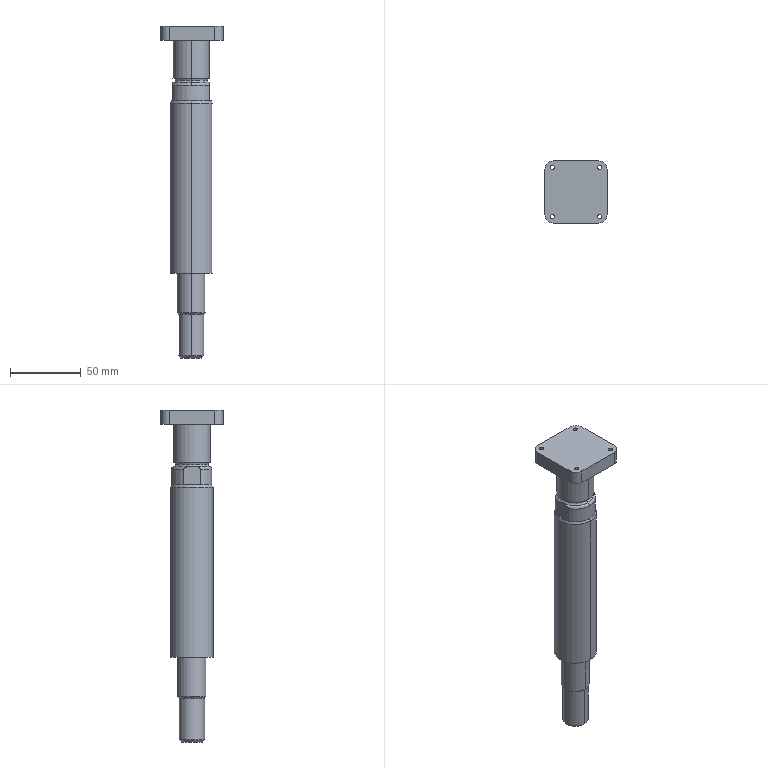Component | SolidWorks | Cylinder-1_PistonRod-2 | 1 solid | 47 faces | volume 145594 mm3 | cylinder 23 | plane 12 | torus 6 | cone 6 | commonest cylinder face diameters 3 x8 12 x4 28.5 x3 30 x2 20 x2 18 x2 26 x2